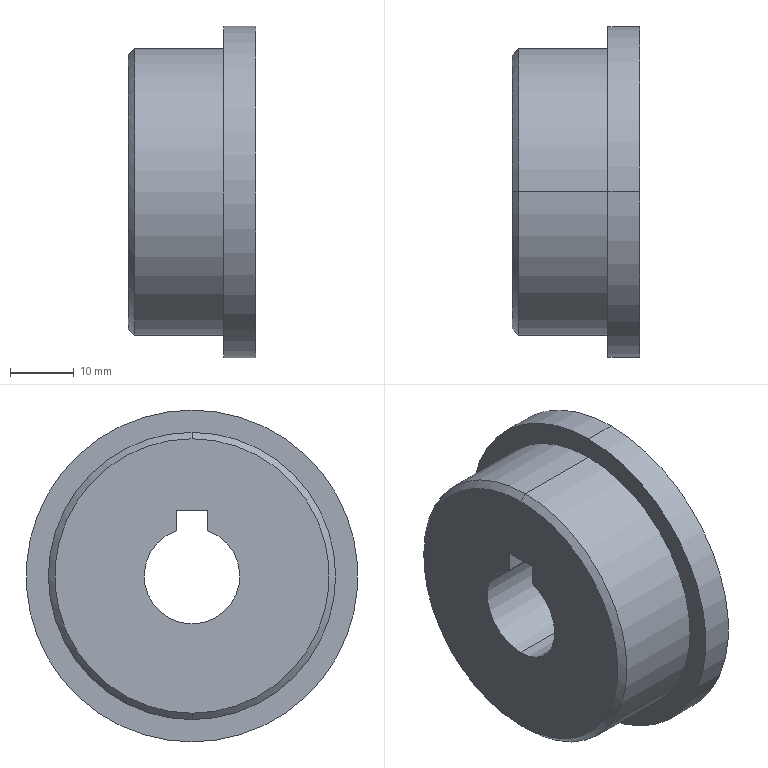Component | SolidWorks | GuideMechanism-1_RollerEndCap01-1 | 1 solid | 14 faces | box 20 x 52 x 52 mm | volume 30577 mm3 | cylinder 6 | plane 6 | cone 2 | commonest cylinder face diameters 52 x2 45 x2 15 x2
build123d program:
from build123d import *

# Parameters (mm, degrees)
SKETCH2_W          = 5
SKETCH2_H          = 4.668
CUT_EXTRUDE1_DEPTH = 42.857
CHAMFER1_SIZE      = 1


with BuildPart() as part:
    # Sketch1 → Revolve1 (revolve)
    with BuildSketch(Plane.XY, mode=Mode.PRIVATE) as revolve1_sk:
        Polygon((7.5, 0), (7.5, 20), (22.5, 20), (22.5, 5), (26, 5), (26, 0), align=None)
    revolve(revolve1_sk.sketch.rotate(Axis((0, 0, 0), (0, 1, 0)), 90), axis=Axis((0, 0, 0), (0, 1, 0)))

    # Sketch2 → Cut-Extrude1 (cut, through all)
    with BuildSketch(Plane.XZ):
        with Locations((0, 7.966)):
            Rectangle(SKETCH2_W, SKETCH2_H)
    extrude(amount=-CUT_EXTRUDE1_DEPTH, mode=Mode.SUBTRACT)

    # Chamfer1
    chamfer1_edges = [part.edges().sort_by_distance(p)[0] for p in [
        (0, 20, 22.5),
    ]]
    chamfer(chamfer1_edges, length=CHAMFER1_SIZE)


solid = part.part

# Placed as in the assembly
solid = solid.moved(Location((-381.772, -352.564, 1209.912), (0, 0, 90)))
STEP:
#1=COLOUR_RGB('',0.7922,0.8196,0.9333);
#2=FILL_AREA_STYLE_COLOUR('',#1);
#3=FILL_AREA_STYLE('',(#2));
#4=SURFACE_STYLE_FILL_AREA(#3);
#5=SURFACE_SIDE_STYLE('',(#4));
#6=SURFACE_STYLE_USAGE(.BOTH.,#5);
#7=PRESENTATION_STYLE_ASSIGNMENT((#6));
#8=CARTESIAN_POINT('',(-15.818,-13.88,48.481));
#9=VERTEX_POINT('',#8);
#10=CARTESIAN_POINT('',(-15.818,-13.88,46.788));
#11=VERTEX_POINT('',#10);
#12=CARTESIAN_POINT('',(-15.818,-13.88,47.634));
#13=DIRECTION('',(-1.,-0.,-0.));
#14=DIRECTION('',(0.,0.,1.));
#15=AXIS2_PLACEMENT_3D('',#12,#13,#14);
#16=CIRCLE('',#15,0.8465);
#17=EDGE_CURVE('',#9,#11,#16,.T.);
#18=ORIENTED_EDGE('',*,*,#17,.F.);
#19=CARTESIAN_POINT('',(-15.778,-13.88,48.52));
#20=VERTEX_POINT('',#19);
#21=CARTESIAN_POINT('',(-15.778,-13.88,48.52));
#22=DIRECTION('',(0.7071,0.,0.7071));
#23=VECTOR('',#22,39.37);
#24=LINE('',#21,#23);
#25=EDGE_CURVE('',#9,#20,#24,.T.);
#26=ORIENTED_EDGE('',*,*,#25,.T.);
#27=CARTESIAN_POINT('',(-15.778,-13.88,46.749));
#28=VERTEX_POINT('',#27);
#29=CARTESIAN_POINT('',(-15.778,-13.88,47.634));
#30=DIRECTION('',(1.,0.,0.));
#31=DIRECTION('',(0.,0.,1.));
#32=AXIS2_PLACEMENT_3D('',#29,#30,#31);
#33=CIRCLE('',#32,0.8858);
#34=EDGE_CURVE('',#28,#20,#33,.T.);
#35=ORIENTED_EDGE('',*,*,#34,.F.);
#36=CARTESIAN_POINT('',(-15.778,-13.88,46.749));
#37=DIRECTION('',(0.7071,-0.,-0.7071));
#38=VECTOR('',#37,39.37);
#39=LINE('',#36,#38);
#40=EDGE_CURVE('',#11,#28,#39,.T.);
#41=ORIENTED_EDGE('',*,*,#40,.F.);
#42=EDGE_LOOP('',(#18,#26,#35,#41));
#43=FACE_OUTER_BOUND('',#42,.T.);
#44=CARTESIAN_POINT('',(-15.778,-13.88,47.634));
#45=DIRECTION('',(1.,0.,0.));
#46=DIRECTION('',(0.,0.,-1.));
#47=AXIS2_PLACEMENT_3D('',#44,#45,#46);
#48=CONICAL_SURFACE('',#47,0.8858,0.7854);
#49=ADVANCED_FACE('',(#43),#48,.T.);
#50=CARTESIAN_POINT('',(-15.227,-13.88,46.611));
#51=VERTEX_POINT('',#50);
#52=CARTESIAN_POINT('',(-15.227,-13.88,48.658));
#53=VERTEX_POINT('',#52);
#54=CARTESIAN_POINT('',(-15.227,-13.88,47.634));
#55=DIRECTION('',(1.,0.,0.));
#56=DIRECTION('',(0.,0.,-1.));
#57=AXIS2_PLACEMENT_3D('',#54,#55,#56);
#58=CIRCLE('',#57,1.024);
#59=EDGE_CURVE('',#51,#53,#58,.T.);
#60=ORIENTED_EDGE('',*,*,#59,.T.);
#61=CARTESIAN_POINT('',(-15.03,-13.88,48.658));
#62=VERTEX_POINT('',#61);
#63=CARTESIAN_POINT('',(-15.03,-13.88,48.658));
#64=DIRECTION('',(1.,0.,0.));
#65=VECTOR('',#64,39.37);
#66=LINE('',#63,#65);
#67=EDGE_CURVE('',#53,#62,#66,.T.);
#68=ORIENTED_EDGE('',*,*,#67,.T.);
#69=CARTESIAN_POINT('',(-15.03,-13.88,46.611));
#70=VERTEX_POINT('',#69);
#71=CARTESIAN_POINT('',(-15.03,-13.88,47.634));
#72=DIRECTION('',(1.,0.,0.));
#73=DIRECTION('',(0.,0.,-1.));
#74=AXIS2_PLACEMENT_3D('',#71,#72,#73);
#75=CIRCLE('',#74,1.024);
#76=EDGE_CURVE('',#70,#62,#75,.T.);
#77=ORIENTED_EDGE('',*,*,#76,.F.);
#78=CARTESIAN_POINT('',(-15.03,-13.88,46.611));
#79=DIRECTION('',(1.,0.,0.));
#80=VECTOR('',#79,39.37);
#81=LINE('',#78,#80);
#82=EDGE_CURVE('',#51,#70,#81,.T.);
#83=ORIENTED_EDGE('',*,*,#82,.F.);
#84=EDGE_LOOP('',(#60,#68,#77,#83));
#85=FACE_OUTER_BOUND('',#84,.T.);
#86=CARTESIAN_POINT('',(-15.03,-13.88,47.634));
#87=DIRECTION('',(1.,0.,0.));
#88=DIRECTION('',(0.,0.,-1.));
#89=AXIS2_PLACEMENT_3D('',#86,#87,#88);
#90=CYLINDRICAL_SURFACE('',#89,1.024);
#91=ADVANCED_FACE('',(#85),#90,.T.);
#92=ORIENTED_EDGE('',*,*,#34,.T.);
#93=CARTESIAN_POINT('',(-15.227,-13.88,48.52));
#94=VERTEX_POINT('',#93);
#95=CARTESIAN_POINT('',(-15.03,-13.88,48.52));
#96=DIRECTION('',(1.,0.,0.));
#97=VECTOR('',#96,39.37);
#98=LINE('',#95,#97);
#99=EDGE_CURVE('',#20,#94,#98,.T.);
#100=ORIENTED_EDGE('',*,*,#99,.T.);
#101=CARTESIAN_POINT('',(-15.227,-13.88,46.749));
#102=VERTEX_POINT('',#101);
#103=CARTESIAN_POINT('',(-15.227,-13.88,47.634));
#104=DIRECTION('',(1.,0.,0.));
#105=DIRECTION('',(0.,0.,-1.));
#106=AXIS2_PLACEMENT_3D('',#103,#104,#105);
#107=CIRCLE('',#106,0.8858);
#108=EDGE_CURVE('',#102,#94,#107,.T.);
#109=ORIENTED_EDGE('',*,*,#108,.F.);
#110=CARTESIAN_POINT('',(-15.03,-13.88,46.749));
#111=DIRECTION('',(1.,0.,0.));
#112=VECTOR('',#111,39.37);
#113=LINE('',#110,#112);
#114=EDGE_CURVE('',#28,#102,#113,.T.);
#115=ORIENTED_EDGE('',*,*,#114,.F.);
#116=EDGE_LOOP('',(#92,#100,#109,#115));
#117=FACE_OUTER_BOUND('',#116,.T.);
#118=CARTESIAN_POINT('',(-15.03,-13.88,47.634));
#119=DIRECTION('',(1.,0.,0.));
#120=DIRECTION('',(0.,0.,-1.));
#121=AXIS2_PLACEMENT_3D('',#118,#119,#120);
#122=CYLINDRICAL_SURFACE('',#121,0.8858);
#123=ADVANCED_FACE('',(#117),#122,.T.);
#124=CARTESIAN_POINT('',(-15.818,-13.88,47.339));
#125=VERTEX_POINT('',#124);
#126=CARTESIAN_POINT('',(-15.818,-13.782,47.913));
#127=VERTEX_POINT('',#126);
#128=CARTESIAN_POINT('',(-15.818,-13.88,47.634));
#129=DIRECTION('',(1.,0.,0.));
#130=DIRECTION('',(0.,0.,-1.));
#131=AXIS2_PLACEMENT_3D('',#128,#129,#130);
#132=CIRCLE('',#131,0.2953);
#133=EDGE_CURVE('',#125,#127,#132,.T.);
#134=ORIENTED_EDGE('',*,*,#133,.F.);
#135=CARTESIAN_POINT('',(-15.03,-13.88,47.339));
#136=VERTEX_POINT('',#135);
#137=CARTESIAN_POINT('',(-15.03,-13.88,47.339));
#138=DIRECTION('',(1.,0.,0.));
#139=VECTOR('',#138,39.37);
#140=LINE('',#137,#139);
#141=EDGE_CURVE('',#125,#136,#140,.T.);
#142=ORIENTED_EDGE('',*,*,#141,.T.);
#143=CARTESIAN_POINT('',(-15.03,-13.782,47.913));
#144=VERTEX_POINT('',#143);
#145=CARTESIAN_POINT('',(-15.03,-13.88,47.634));
#146=DIRECTION('',(1.,0.,0.));
#147=DIRECTION('',(0.,0.,-1.));
#148=AXIS2_PLACEMENT_3D('',#145,#146,#147);
#149=CIRCLE('',#148,0.2953);
#150=EDGE_CURVE('',#136,#144,#149,.T.);
#151=ORIENTED_EDGE('',*,*,#150,.T.);
#152=CARTESIAN_POINT('',(-15.03,-13.782,47.913));
#153=DIRECTION('',(1.,0.,0.));
#154=VECTOR('',#153,39.37);
#155=LINE('',#152,#154);
#156=EDGE_CURVE('',#127,#144,#155,.T.);
#157=ORIENTED_EDGE('',*,*,#156,.F.);
#158=EDGE_LOOP('',(#134,#142,#151,#157));
#159=FACE_OUTER_BOUND('',#158,.T.);
#160=CARTESIAN_POINT('',(-15.03,-13.88,47.634));
#161=DIRECTION('',(1.,0.,0.));
#162=DIRECTION('',(0.,0.,-1.));
#163=AXIS2_PLACEMENT_3D('',#160,#161,#162);
#164=CYLINDRICAL_SURFACE('',#163,0.2953);
#165=ADVANCED_FACE('',(#159),#164,.F.);
#166=CARTESIAN_POINT('',(-15.03,-13.979,48.04));
#167=VERTEX_POINT('',#166);
#168=CARTESIAN_POINT('',(-15.03,-13.979,47.913));
#169=VERTEX_POINT('',#168);
#170=CARTESIAN_POINT('',(-15.03,-13.979,48.04));
#171=DIRECTION('',(0.,0.,-1.));
#172=VECTOR('',#171,39.37);
#173=LINE('',#170,#172);
#174=EDGE_CURVE('',#167,#169,#173,.T.);
#175=ORIENTED_EDGE('',*,*,#174,.F.);
#176=CARTESIAN_POINT('',(-15.03,-13.782,48.04));
#177=VERTEX_POINT('',#176);
#178=CARTESIAN_POINT('',(-15.03,-13.979,48.04));
#179=DIRECTION('',(0.,-1.,0.));
#180=VECTOR('',#179,39.37);
#181=LINE('',#178,#180);
#182=EDGE_CURVE('',#177,#167,#181,.T.);
#183=ORIENTED_EDGE('',*,*,#182,.F.);
#184=CARTESIAN_POINT('',(-15.03,-13.782,48.04));
#185=DIRECTION('',(-0.,-0.,1.));
#186=VECTOR('',#185,39.37);
#187=LINE('',#184,#186);
#188=EDGE_CURVE('',#144,#177,#187,.T.);
#189=ORIENTED_EDGE('',*,*,#188,.F.);
#190=ORIENTED_EDGE('',*,*,#150,.F.);
#191=CARTESIAN_POINT('',(-15.03,-13.88,47.634));
#192=DIRECTION('',(1.,0.,0.));
#193=DIRECTION('',(0.,0.,-1.));
#194=AXIS2_PLACEMENT_3D('',#191,#192,#193);
#195=CIRCLE('',#194,0.2953);
#196=EDGE_CURVE('',#169,#136,#195,.T.);
#197=ORIENTED_EDGE('',*,*,#196,.F.);
#198=EDGE_LOOP('',(#175,#183,#189,#190,#197));
#199=FACE_BOUND('',#198,.T.);
#200=ORIENTED_EDGE('',*,*,#76,.T.);
#201=CARTESIAN_POINT('',(-15.03,-13.88,47.634));
#202=DIRECTION('',(1.,0.,0.));
#203=DIRECTION('',(0.,0.,-1.));
#204=AXIS2_PLACEMENT_3D('',#201,#202,#203);
#205=CIRCLE('',#204,1.024);
#206=EDGE_CURVE('',#62,#70,#205,.T.);
#207=ORIENTED_EDGE('',*,*,#206,.T.);
#208=EDGE_LOOP('',(#200,#207));
#209=FACE_OUTER_BOUND('',#208,.T.);
#210=CARTESIAN_POINT('',(-15.03,-12.857,47.634));
#211=DIRECTION('',(1.,0.,0.));
#212=DIRECTION('',(0.,-0.,-1.));
#213=AXIS2_PLACEMENT_3D('',#210,#211,#212);
#214=PLANE('',#213);
#215=ADVANCED_FACE('',(#199,#209),#214,.T.);
#216=ORIENTED_EDGE('',*,*,#141,.F.);
#217=CARTESIAN_POINT('',(-15.818,-13.979,47.913));
#218=VERTEX_POINT('',#217);
#219=CARTESIAN_POINT('',(-15.818,-13.88,47.634));
#220=DIRECTION('',(1.,0.,0.));
#221=DIRECTION('',(0.,0.,-1.));
#222=AXIS2_PLACEMENT_3D('',#219,#220,#221);
#223=CIRCLE('',#222,0.2953);
#224=EDGE_CURVE('',#218,#125,#223,.T.);
#225=ORIENTED_EDGE('',*,*,#224,.F.);
#226=CARTESIAN_POINT('',(-15.03,-13.979,47.913));
#227=DIRECTION('',(-1.,-0.,-0.));
#228=VECTOR('',#227,39.37);
#229=LINE('',#226,#228);
#230=EDGE_CURVE('',#169,#218,#229,.T.);
#231=ORIENTED_EDGE('',*,*,#230,.F.);
#232=ORIENTED_EDGE('',*,*,#196,.T.);
#233=EDGE_LOOP('',(#216,#225,#231,#232));
#234=FACE_OUTER_BOUND('',#233,.T.);
#235=CARTESIAN_POINT('',(-15.03,-13.88,47.634));
#236=DIRECTION('',(1.,0.,0.));
#237=DIRECTION('',(0.,0.,-1.));
#238=AXIS2_PLACEMENT_3D('',#235,#236,#237);
#239=CYLINDRICAL_SURFACE('',#238,0.2953);
#240=ADVANCED_FACE('',(#234),#239,.F.);
#241=CARTESIAN_POINT('',(-15.818,-13.88,47.634));
#242=DIRECTION('',(-1.,-0.,-0.));
#243=DIRECTION('',(0.,0.,1.));
#244=AXIS2_PLACEMENT_3D('',#241,#242,#243);
#245=CIRCLE('',#244,0.8465);
#246=EDGE_CURVE('',#11,#9,#245,.T.);
#247=ORIENTED_EDGE('',*,*,#246,.T.);
#248=ORIENTED_EDGE('',*,*,#17,.T.);
#249=EDGE_LOOP('',(#247,#248));
#250=FACE_OUTER_BOUND('',#249,.T.);
#251=CARTESIAN_POINT('',(-15.818,-13.979,48.04));
#252=VERTEX_POINT('',#251);
#253=CARTESIAN_POINT('',(-15.818,-13.979,48.04));
#254=DIRECTION('',(0.,0.,-1.));
#255=VECTOR('',#254,39.37);
#256=LINE('',#253,#255);
#257=EDGE_CURVE('',#252,#218,#256,.T.);
#258=ORIENTED_EDGE('',*,*,#257,.T.);
#259=ORIENTED_EDGE('',*,*,#224,.T.);
#260=ORIENTED_EDGE('',*,*,#133,.T.);
#261=CARTESIAN_POINT('',(-15.818,-13.782,48.04));
#262=VERTEX_POINT('',#261);
#263=CARTESIAN_POINT('',(-15.818,-13.782,47.634));
#264=DIRECTION('',(0.,0.,-1.));
#265=VECTOR('',#264,39.37);
#266=LINE('',#263,#265);
#267=EDGE_CURVE('',#262,#127,#266,.T.);
#268=ORIENTED_EDGE('',*,*,#267,.F.);
#269=CARTESIAN_POINT('',(-15.818,-13.979,48.04));
#270=DIRECTION('',(0.,-1.,0.));
#271=VECTOR('',#270,39.37);
#272=LINE('',#269,#271);
#273=EDGE_CURVE('',#262,#252,#272,.T.);
#274=ORIENTED_EDGE('',*,*,#273,.T.);
#275=EDGE_LOOP('',(#258,#259,#260,#268,#274));
#276=FACE_BOUND('',#275,.T.);
#277=CARTESIAN_POINT('',(-15.818,-13.585,47.634));
#278=DIRECTION('',(-1.,-0.,-0.));
#279=DIRECTION('',(-0.,0.,1.));
#280=AXIS2_PLACEMENT_3D('',#277,#278,#279);
#281=PLANE('',#280);
#282=ADVANCED_FACE('',(#250,#276),#281,.T.);
#283=ORIENTED_EDGE('',*,*,#99,.F.);
#284=CARTESIAN_POINT('',(-15.778,-13.88,47.634));
#285=DIRECTION('',(1.,0.,0.));
#286=DIRECTION('',(0.,0.,1.));
#287=AXIS2_PLACEMENT_3D('',#284,#285,#286);
#288=CIRCLE('',#287,0.8858);
#289=EDGE_CURVE('',#20,#28,#288,.T.);
#290=ORIENTED_EDGE('',*,*,#289,.T.);
#291=ORIENTED_EDGE('',*,*,#114,.T.);
#292=CARTESIAN_POINT('',(-15.227,-13.88,47.634));
#293=DIRECTION('',(1.,0.,0.));
#294=DIRECTION('',(0.,0.,-1.));
#295=AXIS2_PLACEMENT_3D('',#292,#293,#294);
#296=CIRCLE('',#295,0.8858);
#297=EDGE_CURVE('',#94,#102,#296,.T.);
#298=ORIENTED_EDGE('',*,*,#297,.F.);
#299=EDGE_LOOP('',(#283,#290,#291,#298));
#300=FACE_OUTER_BOUND('',#299,.T.);
#301=CARTESIAN_POINT('',(-15.03,-13.88,47.634));
#302=DIRECTION('',(1.,0.,0.));
#303=DIRECTION('',(0.,0.,-1.));
#304=AXIS2_PLACEMENT_3D('',#301,#302,#303);
#305=CYLINDRICAL_SURFACE('',#304,0.8858);
#306=ADVANCED_FACE('',(#300),#305,.T.);
#307=ORIENTED_EDGE('',*,*,#108,.T.);
#308=ORIENTED_EDGE('',*,*,#297,.T.);
#309=EDGE_LOOP('',(#307,#308));
#310=FACE_BOUND('',#309,.T.);
#311=ORIENTED_EDGE('',*,*,#59,.F.);
#312=CARTESIAN_POINT('',(-15.227,-13.88,47.634));
#313=DIRECTION('',(1.,0.,0.));
#314=DIRECTION('',(0.,0.,-1.));
#315=AXIS2_PLACEMENT_3D('',#312,#313,#314);
#316=CIRCLE('',#315,1.024);
#317=EDGE_CURVE('',#53,#51,#316,.T.);
#318=ORIENTED_EDGE('',*,*,#317,.F.);
#319=EDGE_LOOP('',(#311,#318));
#320=FACE_OUTER_BOUND('',#319,.T.);
#321=CARTESIAN_POINT('',(-15.227,-12.995,47.634));
#322=DIRECTION('',(-1.,-0.,-0.));
#323=DIRECTION('',(-0.,0.,1.));
#324=AXIS2_PLACEMENT_3D('',#321,#322,#323);
#325=PLANE('',#324);
#326=ADVANCED_FACE('',(#310,#320),#325,.T.);
#327=ORIENTED_EDGE('',*,*,#67,.F.);
#328=ORIENTED_EDGE('',*,*,#317,.T.);
#329=ORIENTED_EDGE('',*,*,#82,.T.);
#330=ORIENTED_EDGE('',*,*,#206,.F.);
#331=EDGE_LOOP('',(#327,#328,#329,#330));
#332=FACE_OUTER_BOUND('',#331,.T.);
#333=CARTESIAN_POINT('',(-15.03,-13.88,47.634));
#334=DIRECTION('',(1.,0.,0.));
#335=DIRECTION('',(0.,0.,-1.));
#336=AXIS2_PLACEMENT_3D('',#333,#334,#335);
#337=CYLINDRICAL_SURFACE('',#336,1.024);
#338=ADVANCED_FACE('',(#332),#337,.T.);
#339=ORIENTED_EDGE('',*,*,#230,.T.);
#340=ORIENTED_EDGE('',*,*,#257,.F.);
#341=CARTESIAN_POINT('',(-15.818,-13.979,48.04));
#342=DIRECTION('',(1.,0.,0.));
#343=VECTOR('',#342,39.37);
#344=LINE('',#341,#343);
#345=EDGE_CURVE('',#252,#167,#344,.T.);
#346=ORIENTED_EDGE('',*,*,#345,.T.);
#347=ORIENTED_EDGE('',*,*,#174,.T.);
#348=EDGE_LOOP('',(#339,#340,#346,#347));
#349=FACE_OUTER_BOUND('',#348,.T.);
#350=CARTESIAN_POINT('',(-15.818,-13.979,48.04));
#351=DIRECTION('',(0.,-1.,-0.));
#352=DIRECTION('',(-0.,-0.,1.));
#353=AXIS2_PLACEMENT_3D('',#350,#351,#352);
#354=PLANE('',#353);
#355=ADVANCED_FACE('',(#349),#354,.F.);
#356=ORIENTED_EDGE('',*,*,#182,.T.);
#357=ORIENTED_EDGE('',*,*,#345,.F.);
#358=ORIENTED_EDGE('',*,*,#273,.F.);
#359=CARTESIAN_POINT('',(-15.818,-13.782,48.04));
#360=DIRECTION('',(1.,0.,0.));
#361=VECTOR('',#360,39.37);
#362=LINE('',#359,#361);
#363=EDGE_CURVE('',#262,#177,#362,.T.);
#364=ORIENTED_EDGE('',*,*,#363,.T.);
#365=EDGE_LOOP('',(#356,#357,#358,#364));
#366=FACE_OUTER_BOUND('',#365,.T.);
#367=CARTESIAN_POINT('',(-15.818,-13.979,48.04));
#368=DIRECTION('',(-0.,0.,1.));
#369=DIRECTION('',(-0.,1.,-0.));
#370=AXIS2_PLACEMENT_3D('',#367,#368,#369);
#371=PLANE('',#370);
#372=ADVANCED_FACE('',(#366),#371,.F.);
#373=ORIENTED_EDGE('',*,*,#156,.T.);
#374=ORIENTED_EDGE('',*,*,#188,.T.);
#375=ORIENTED_EDGE('',*,*,#363,.F.);
#376=ORIENTED_EDGE('',*,*,#267,.T.);
#377=EDGE_LOOP('',(#373,#374,#375,#376));
#378=FACE_OUTER_BOUND('',#377,.T.);
#379=CARTESIAN_POINT('',(-15.818,-13.782,48.04));
#380=DIRECTION('',(-0.,1.,0.));
#381=DIRECTION('',(0.,0.,-1.));
#382=AXIS2_PLACEMENT_3D('',#379,#380,#381);
#383=PLANE('',#382);
#384=ADVANCED_FACE('',(#378),#383,.F.);
#385=ORIENTED_EDGE('',*,*,#25,.F.);
#386=ORIENTED_EDGE('',*,*,#246,.F.);
#387=ORIENTED_EDGE('',*,*,#40,.T.);
#388=ORIENTED_EDGE('',*,*,#289,.F.);
#389=EDGE_LOOP('',(#385,#386,#387,#388));
#390=FACE_OUTER_BOUND('',#389,.T.);
#391=CARTESIAN_POINT('',(-15.778,-13.88,47.634));
#392=DIRECTION('',(1.,0.,0.));
#393=DIRECTION('',(0.,0.,-1.));
#394=AXIS2_PLACEMENT_3D('',#391,#392,#393);
#395=CONICAL_SURFACE('',#394,0.8858,0.7854);
#396=ADVANCED_FACE('',(#390),#395,.T.);
#397=CLOSED_SHELL('',(#49,#91,#123,#165,#215,#240,#282,#306,#326,#338,#355,#372,#384,#396));
#398=MANIFOLD_SOLID_BREP('',#397);
#399=STYLED_ITEM('',(#7),#398);
#400=(LENGTH_UNIT()NAMED_UNIT(*)SI_UNIT($,.METRE.));
#401=LENGTH_MEASURE_WITH_UNIT(LENGTH_MEASURE(0.0254),#400);
#402=DIMENSIONAL_EXPONENTS(1.,0.,0.,0.,0.,0.,0.);
#403=(CONVERSION_BASED_UNIT('',#401)LENGTH_UNIT()NAMED_UNIT(#402));
#404=UNCERTAINTY_MEASURE_WITH_UNIT(LENGTH_MEASURE(0.00001),#403,'','');
#405=(NAMED_UNIT(*)PLANE_ANGLE_UNIT()SI_UNIT($,.RADIAN.));
#406=(NAMED_UNIT(*)SI_UNIT($,.STERADIAN.)SOLID_ANGLE_UNIT());
#407=(GEOMETRIC_REPRESENTATION_CONTEXT(3)GLOBAL_UNCERTAINTY_ASSIGNED_CONTEXT((#404))GLOBAL_UNIT_ASSIGNED_CONTEXT((#403,#405,#406))REPRESENTATION_CONTEXT('',''));
#408=MECHANICAL_DESIGN_GEOMETRIC_PRESENTATION_REPRESENTATION('',(#399),#407);
#409=PRESENTATION_LAYER_ASSIGNMENT('','',(#399));
#410=CARTESIAN_POINT('',(0.,0.,0.));
#411=DIRECTION('',(0.,0.,1.));
#412=DIRECTION('',(1.,0.,0.));
#413=AXIS2_PLACEMENT_3D('',#410,#411,#412);
#414=(LENGTH_UNIT()NAMED_UNIT(*)SI_UNIT($,.METRE.));
#415=LENGTH_MEASURE_WITH_UNIT(LENGTH_MEASURE(0.0254),#414);
#416=DIMENSIONAL_EXPONENTS(1.,0.,0.,0.,0.,0.,0.);
#417=(CONVERSION_BASED_UNIT('',#415)LENGTH_UNIT()NAMED_UNIT(#416));
#418=UNCERTAINTY_MEASURE_WITH_UNIT(LENGTH_MEASURE(0.00001),#417,'','');
#419=(NAMED_UNIT(*)PLANE_ANGLE_UNIT()SI_UNIT($,.RADIAN.));
#420=(NAMED_UNIT(*)SI_UNIT($,.STERADIAN.)SOLID_ANGLE_UNIT());
#421=(GEOMETRIC_REPRESENTATION_CONTEXT(3)GLOBAL_UNCERTAINTY_ASSIGNED_CONTEXT((#418))GLOBAL_UNIT_ASSIGNED_CONTEXT((#417,#419,#420))REPRESENTATION_CONTEXT('',''));
#422=ADVANCED_BREP_SHAPE_REPRESENTATION('',(#398,#413),#421);